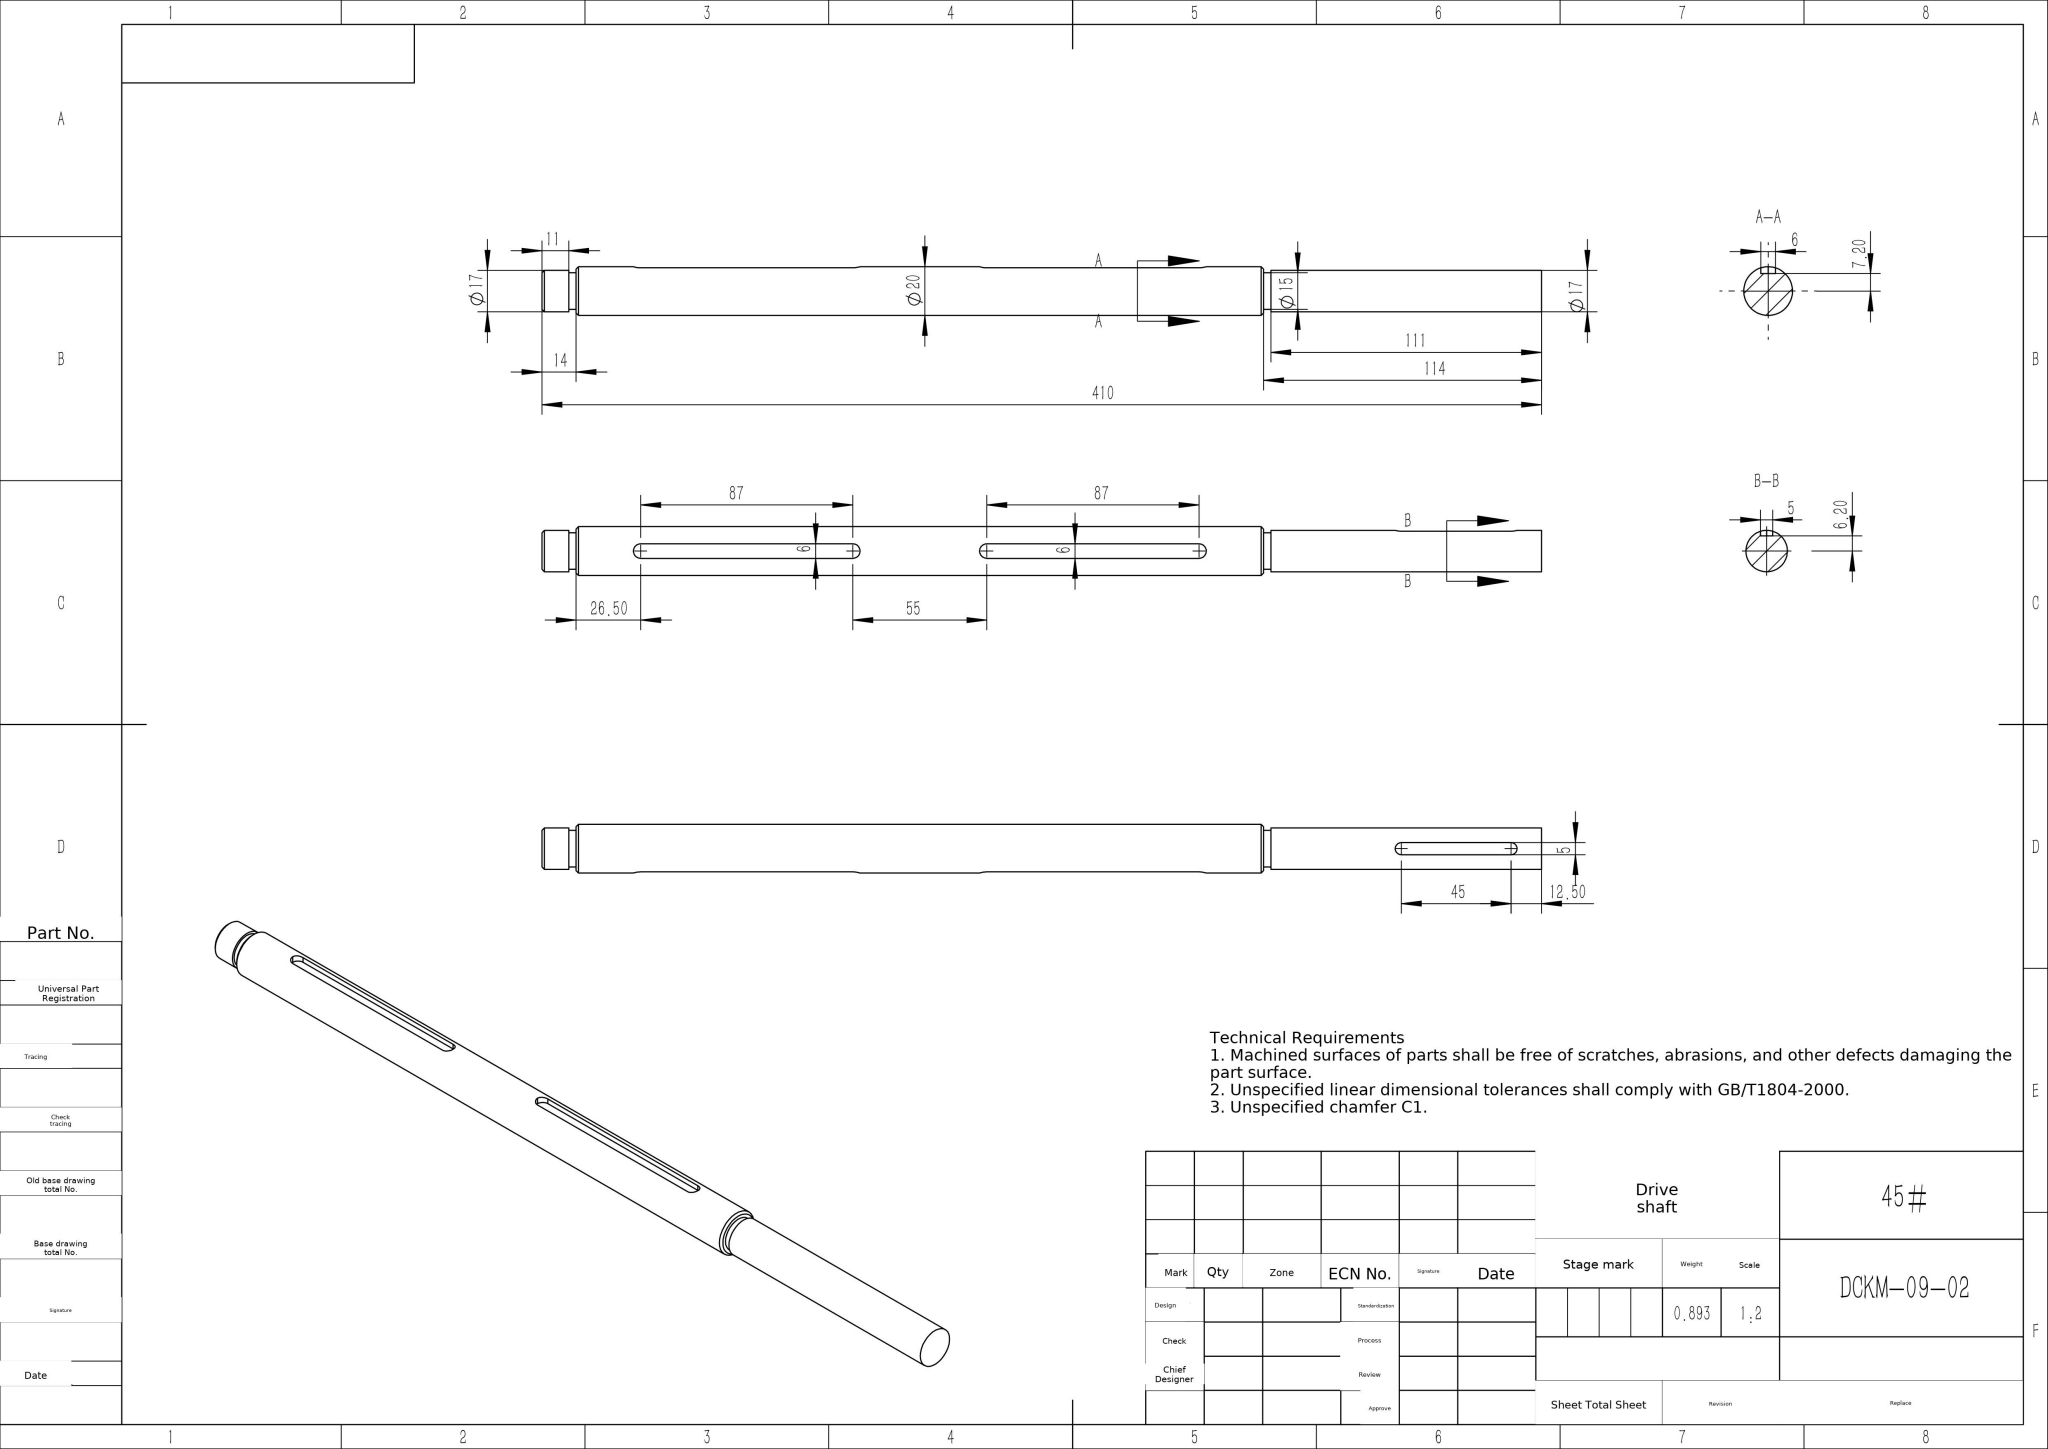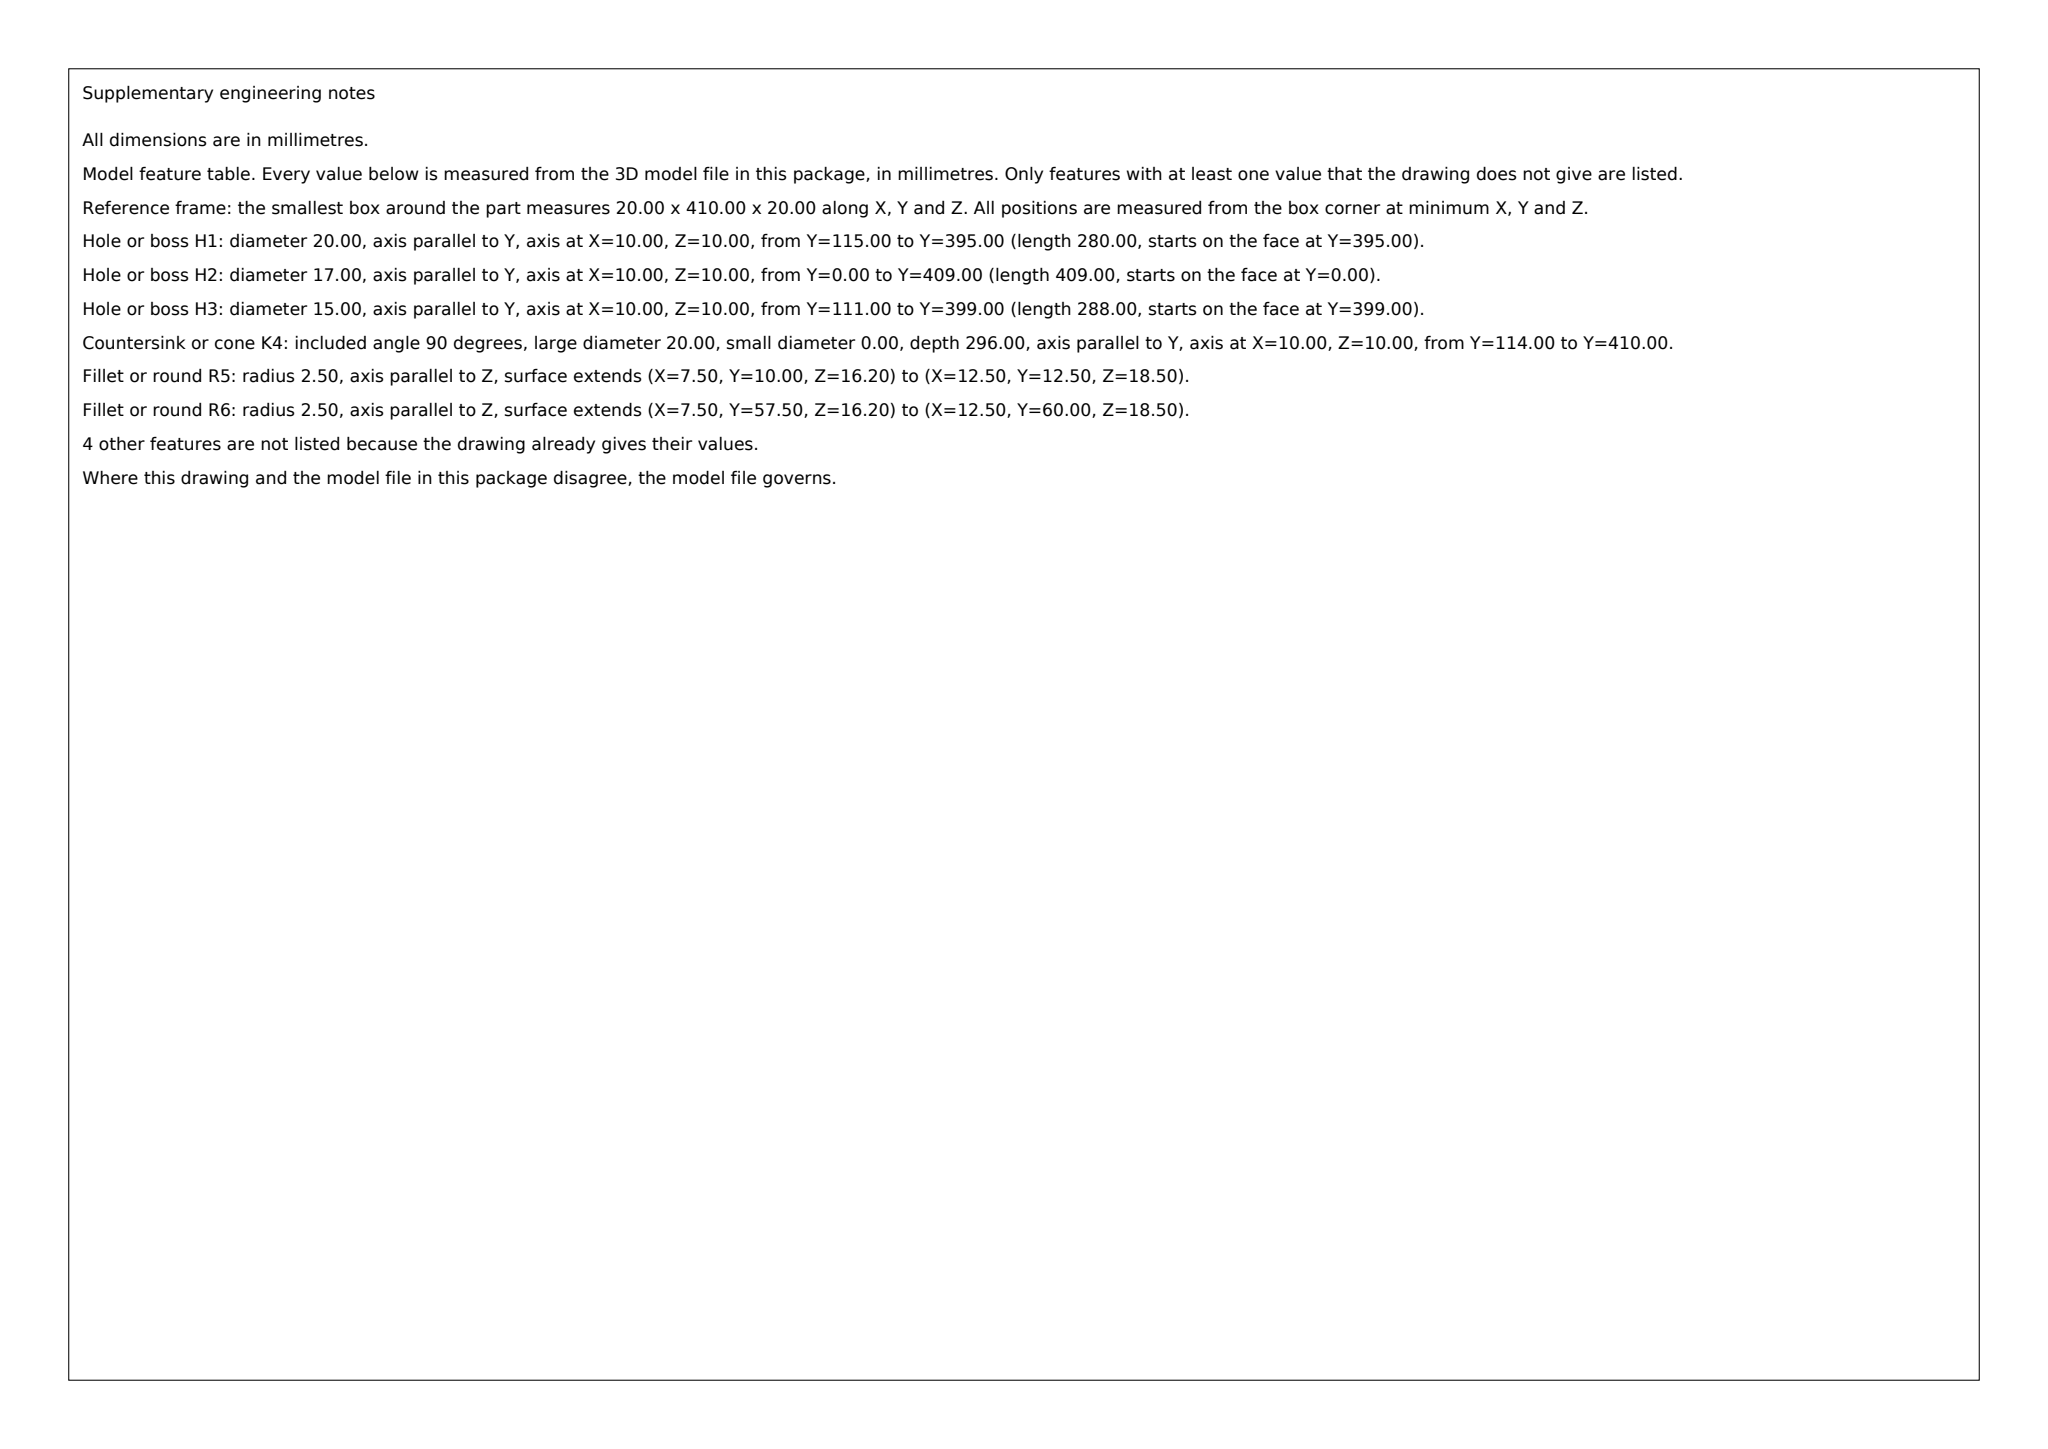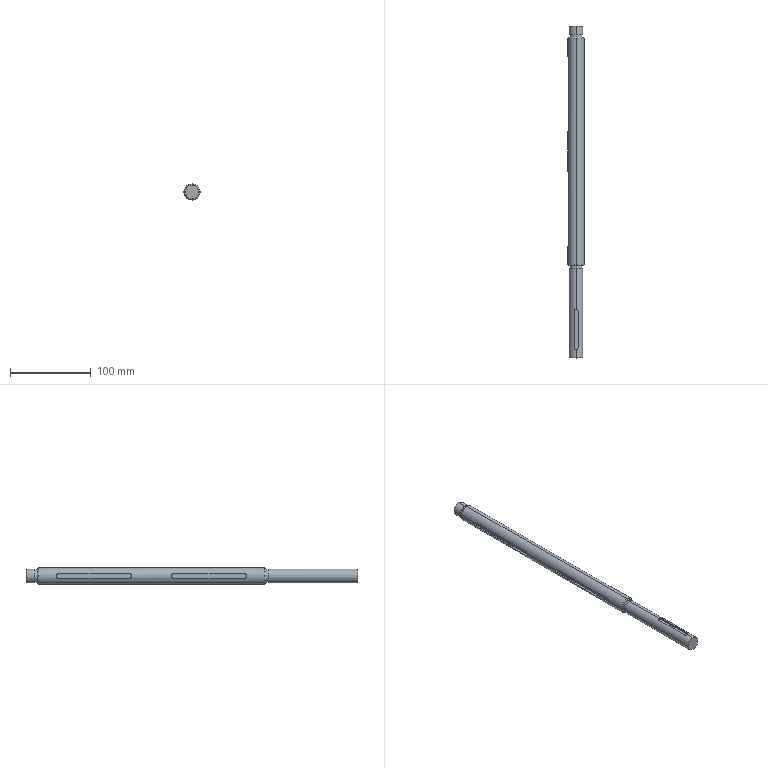Part | SolidWorks | mm | material 45# | 1 solid | 43 faces | box 20 x 410 x 20 mm | volume 113809 mm3 | cylinder 22 | plane 15 | cone 6 | commonest cylinder face diameters 6 x8 17 x4 15 x4 5 x4 20 x2